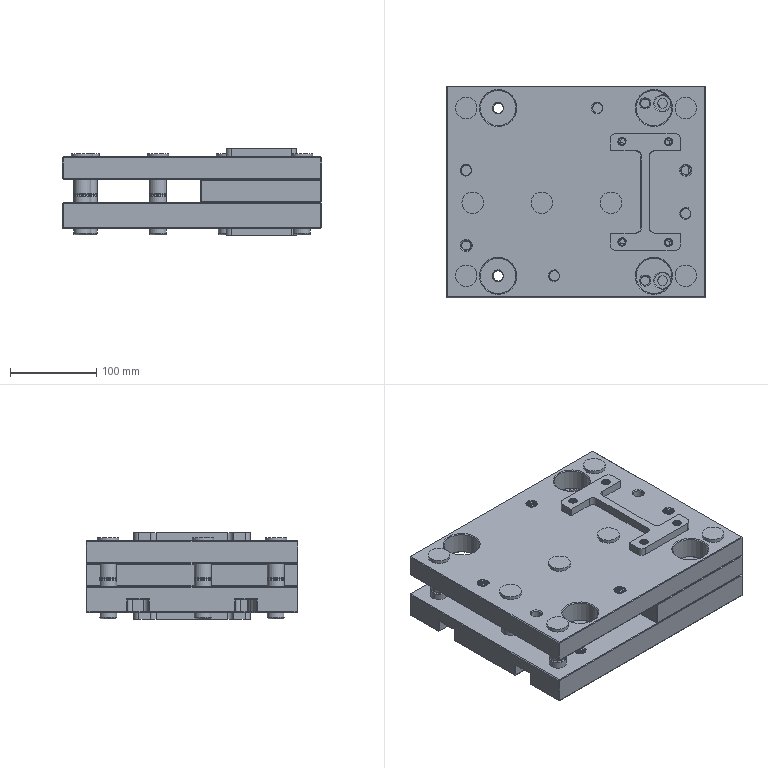Assembly | NX | mm | 11 component files | 11 solids | 525 faces | box 300 x 245 x 100 mm | volume 4792697 mm3 | plane 220 | cylinder 158 | torus 70 | cone 43 | spline 34 | commonest cylinder face diameters 20.015 x42 12 x19 14 x8 11.985 x8 25 x7 12.015 x7 1.015 x7 11 x6
Bill of materials:
unnamed part 1 | 1 |  | Flat rectangular plate with an I-shaped through-cutout near one side, several plain round through holes, and four small threaded holes.
unnamed part 2 | 1 |  | Thicker rectangular block-plate with a central I-shaped through-cutout, counterbored and plain holes at both ends, and a shallow rounded-end slot along one long edge.
unnamed part 3 | 1 |  | Flat rectangular plate with an I-shaped through-cutout, four large corner bores, several medium and small through holes, and small threaded or blind holes.
unnamed part 4 | 1 |  | Straight prismatic block with an I-shaped cross-section, rounded fillets and corners, and small threaded holes in the flange ends.
unnamed part 5 | 7 |  | Cylindrical pin with a thin larger-diameter head at one end and three shallow grooves around the shank.
Mates:
1. fix | punch_holder 1 component
2. center | piller_bush 7 face | piller_bush 7 face | punch_holder 1 face
3. distance | punch_holder 1 face | piller_bush 7 face
4. center | piller_bush 6 face | piller_bush 6 face | punch_holder 1 face
5. distance | punch_holder 1 face | piller_bush 6 face
6. center | piller_bush 5 face | piller_bush 5 face | punch_holder 1 face
7. distance | punch_holder 1 face | piller_bush 5 face
8. center | piller_bush 4 face | piller_bush 4 face | punch_holder 1 face
9. distance | punch_holder 1 face | piller_bush 4 face
10. concentric | die 1 edge | punch_holder 1 edge
11. concentric | stripper 1 edge | die 1 edge
12. distance | punch 1 face | punch_holder 1 face
13. distance | punch 1 face | punch_holder 1 face
14. distance | punch 1 face | stripper 1 face
15. center | punch_holder 1 face | stripper 1 face | piller_bush 3 face
16. distance | punch_holder 1 face | piller_bush 3 face
17. center | punch_holder 1 face | stripper 1 face | piller_bush 2 face
18. distance | punch_holder 1 face | piller_bush 2 face
19. center | piller_bush 1 face | punch_holder 1 face | stripper 1 face
20. distance | punch_holder 1 face | piller_bush 1 face